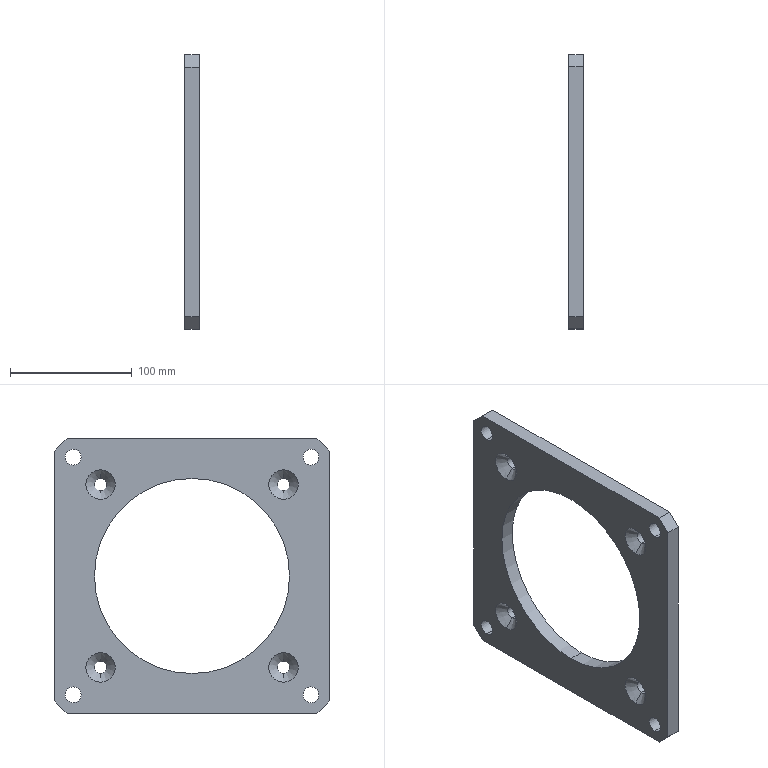CAM job | Mastercam | mm | 9 operations | part box 12 x 225 x 225
1. Facing | 24 - 100 平铣刀
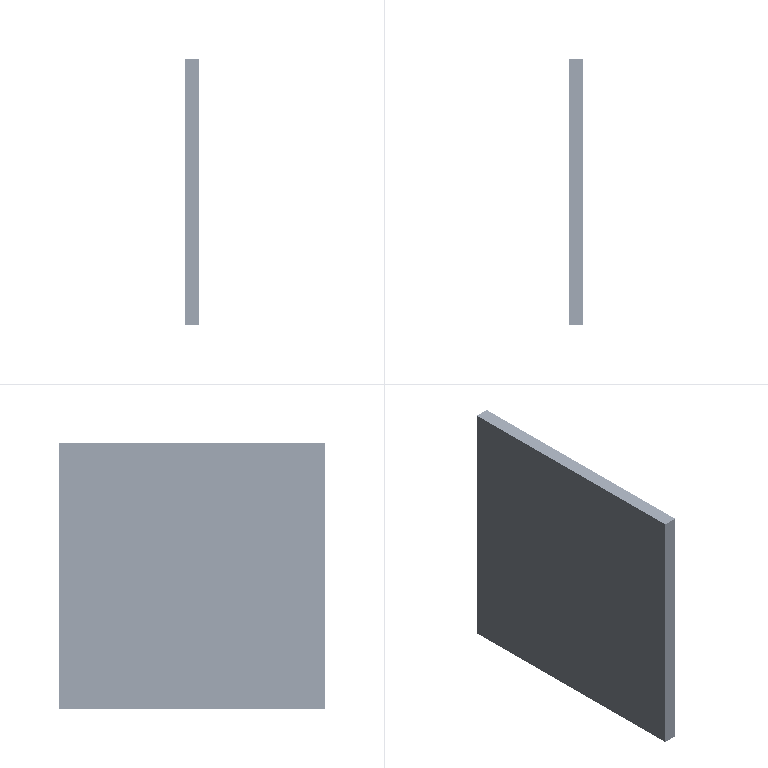2. Contour (Ramp) | 10 - 10 平铣刀
3. Contour (2D) | 10 - 10 平铣刀
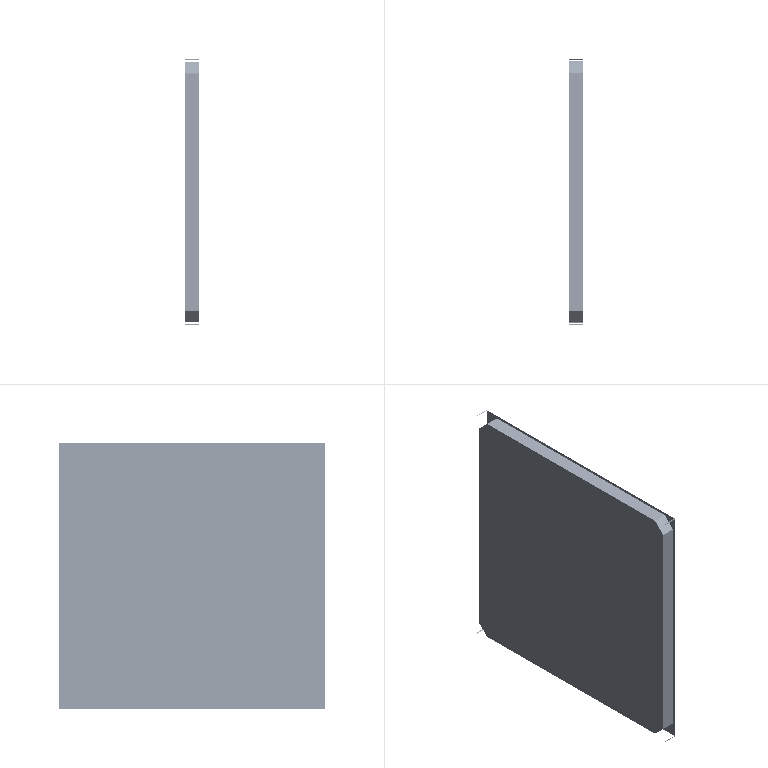4. Contour (2D chamfer) | 7 - 4 倒角刀
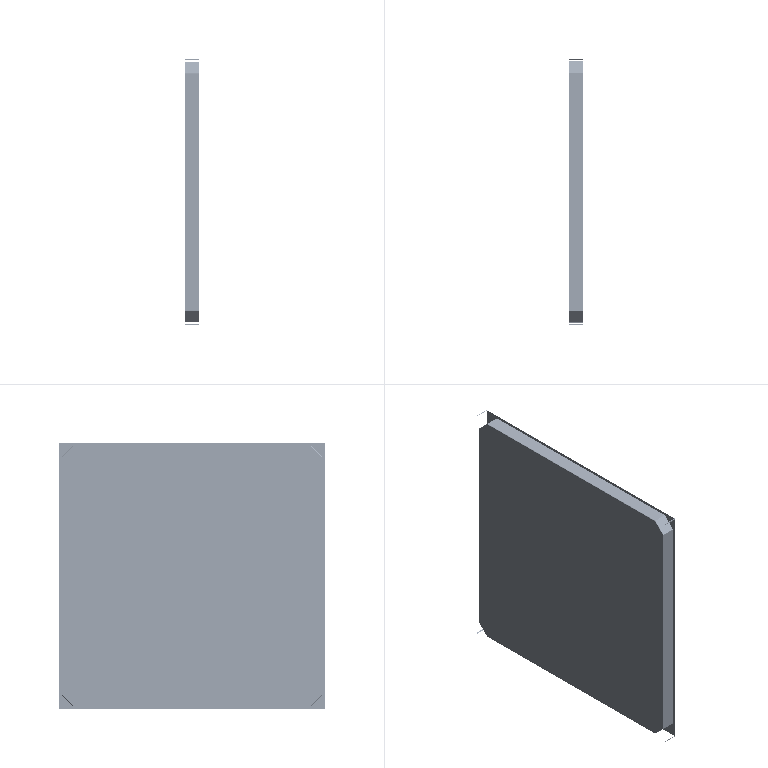5. Contour (Ramp) | 4 - 4 平铣刀
6. Contour (Ramp) | 3 - 3 平铣刀
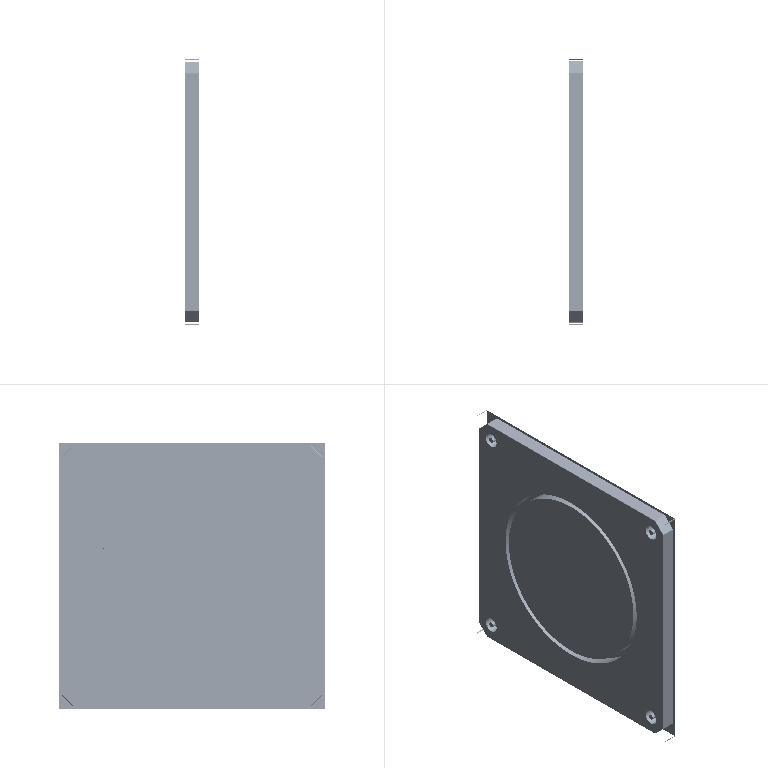7. Contour (2D chamfer) | 7 - 4 倒角刀
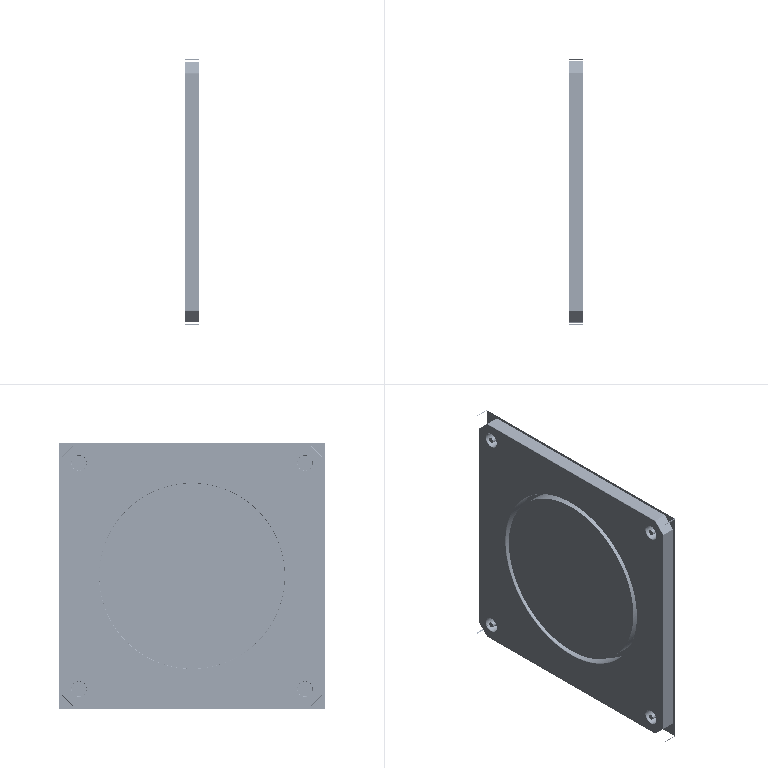8. Contour (Ramp) | 5 - 5 平铣刀
9. 3D High Speed (Waterline) | 9 - 8 圆鼻铣刀